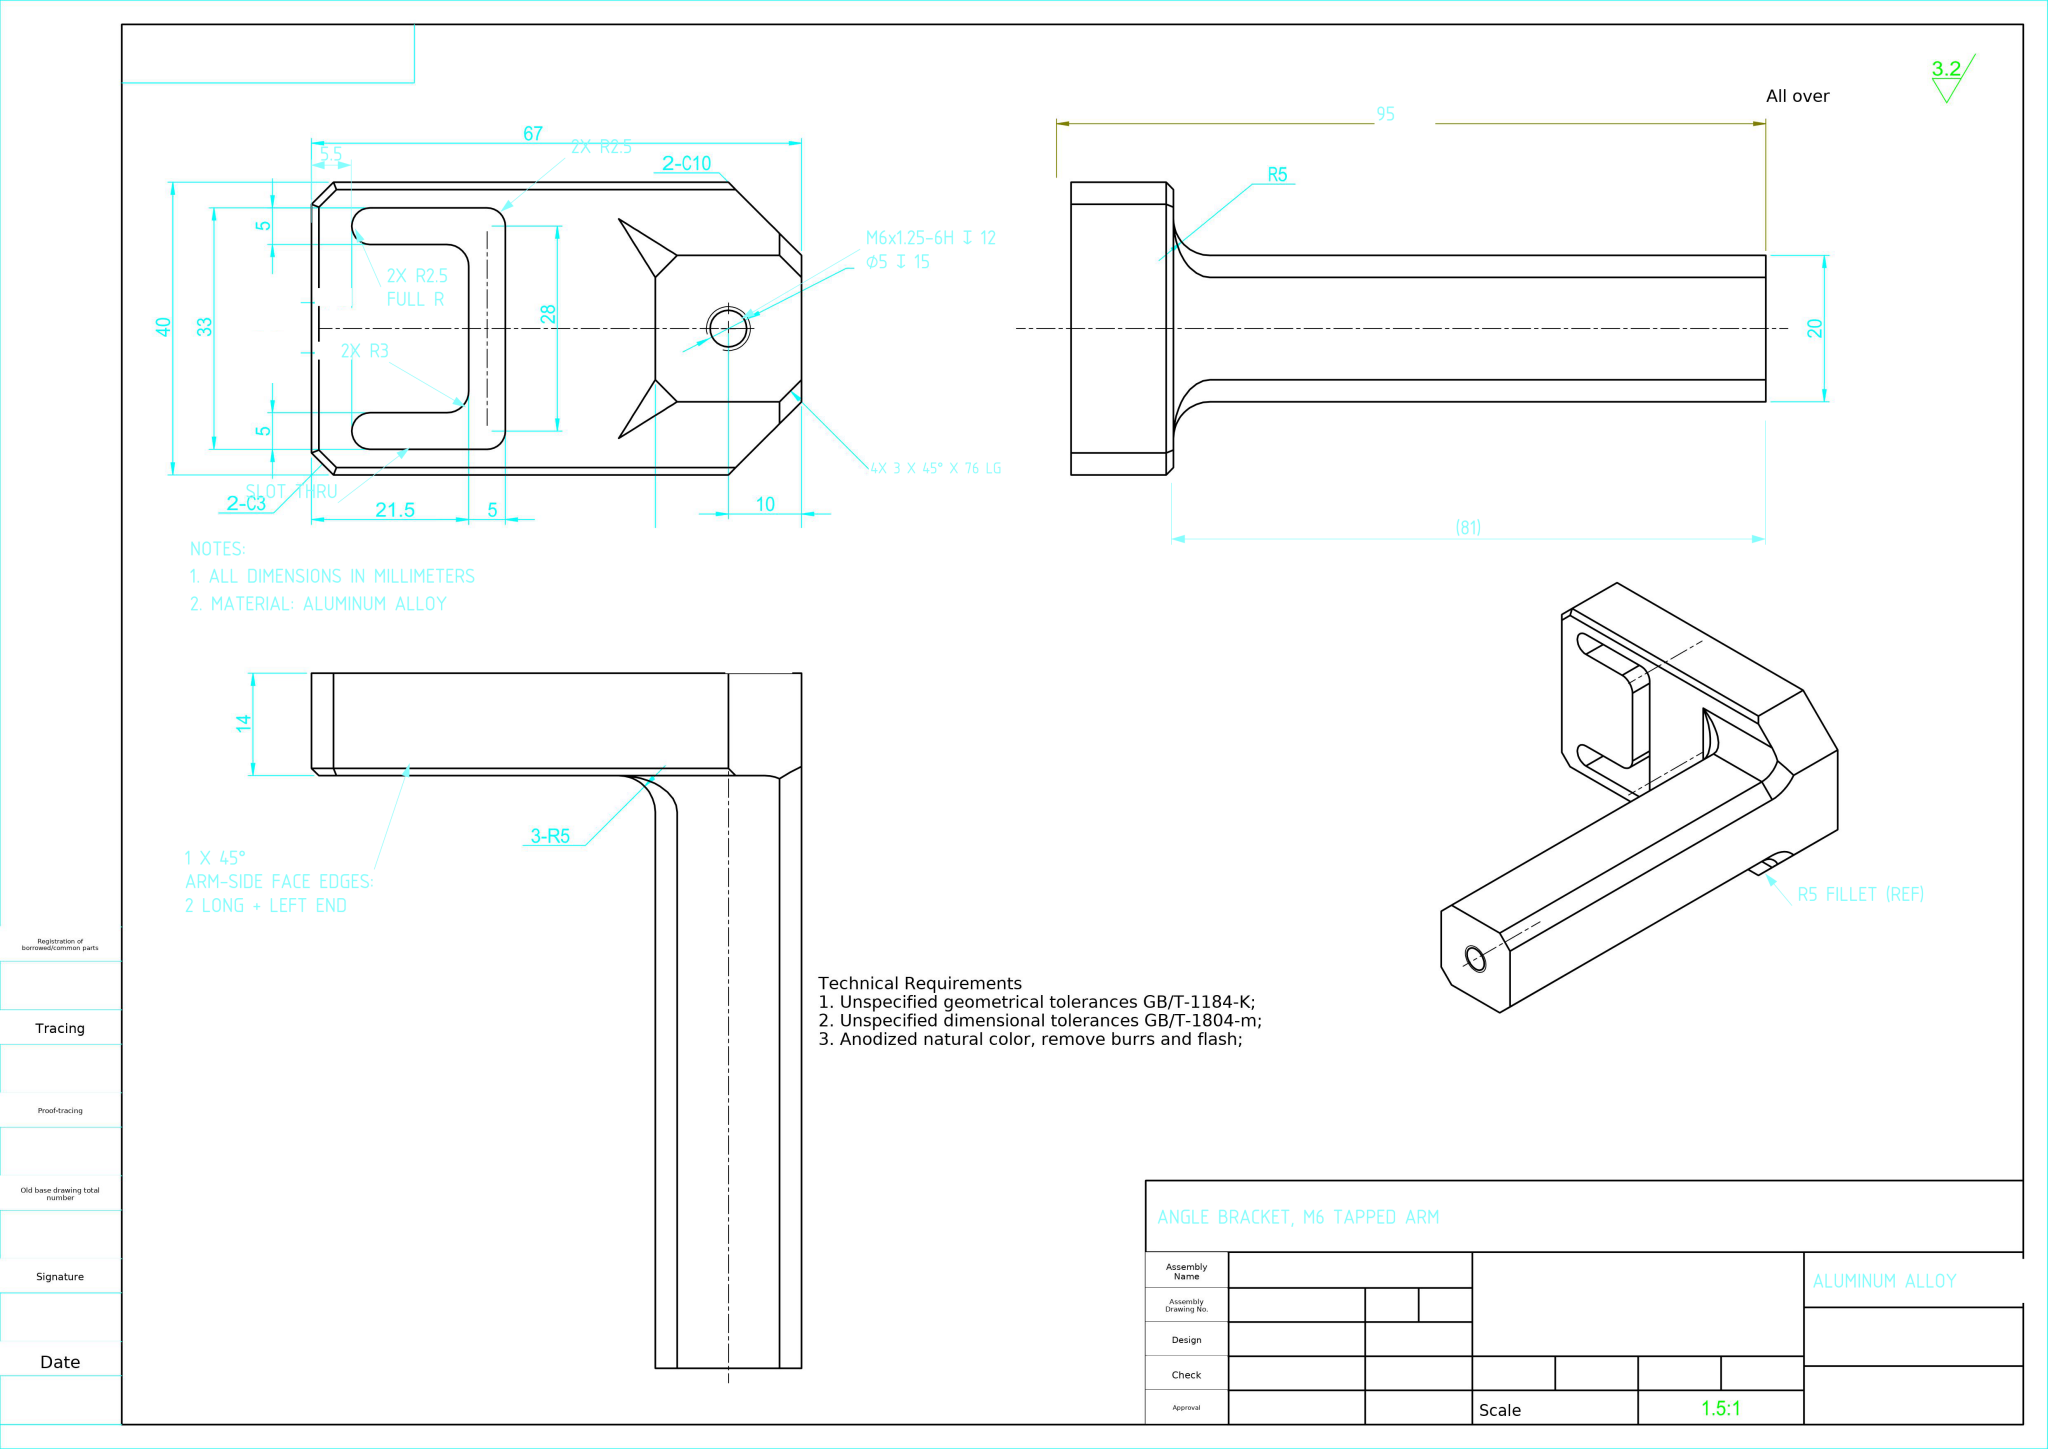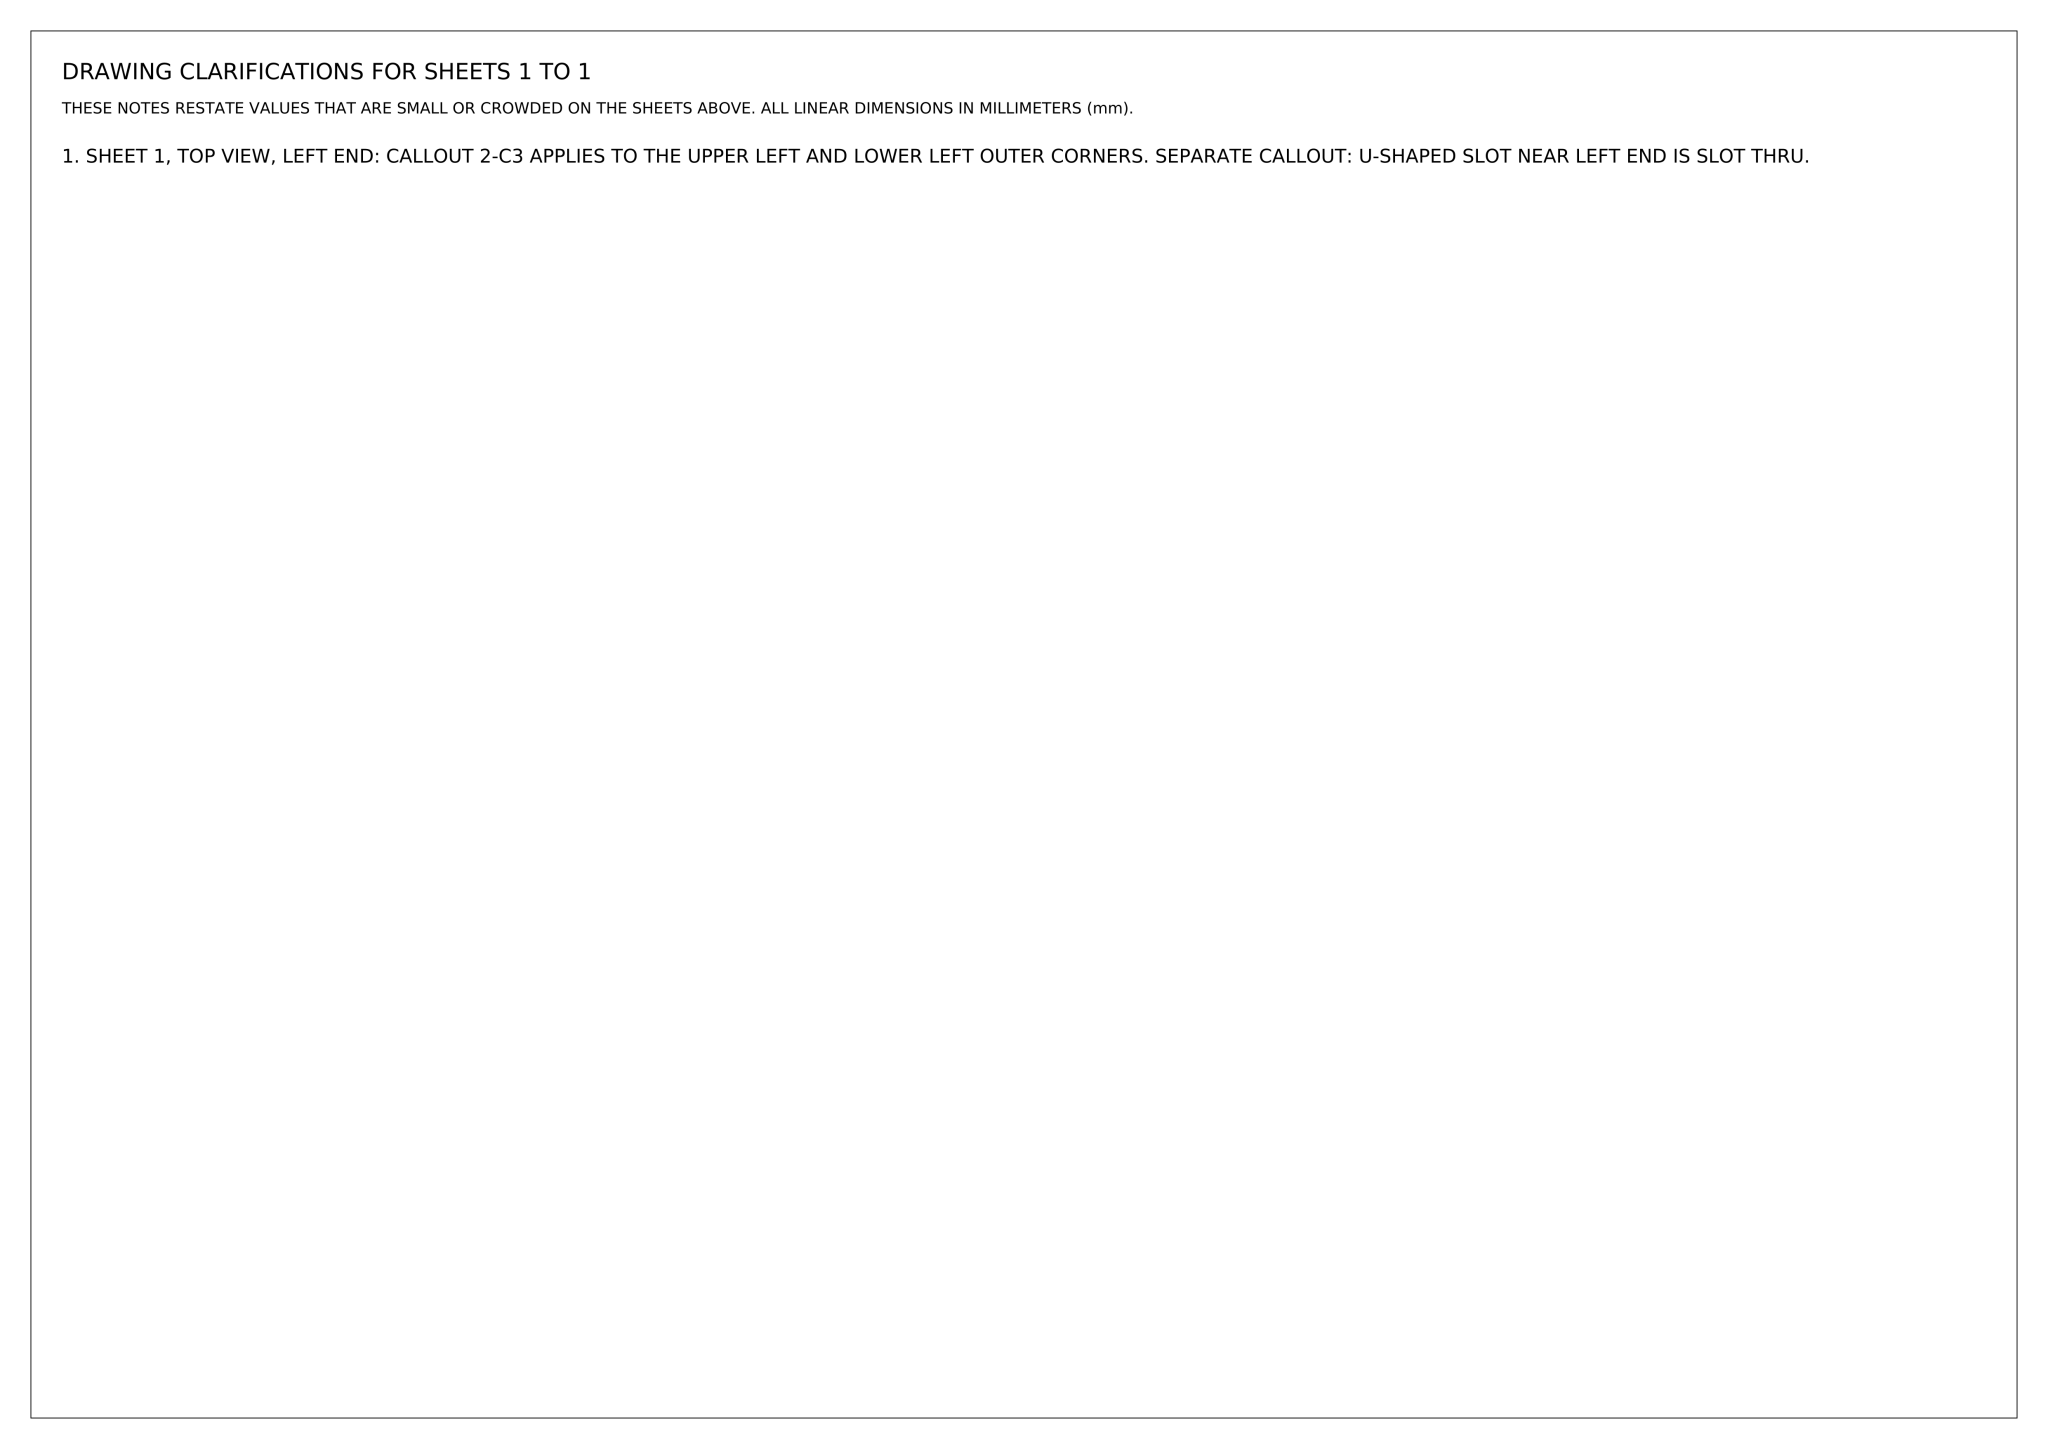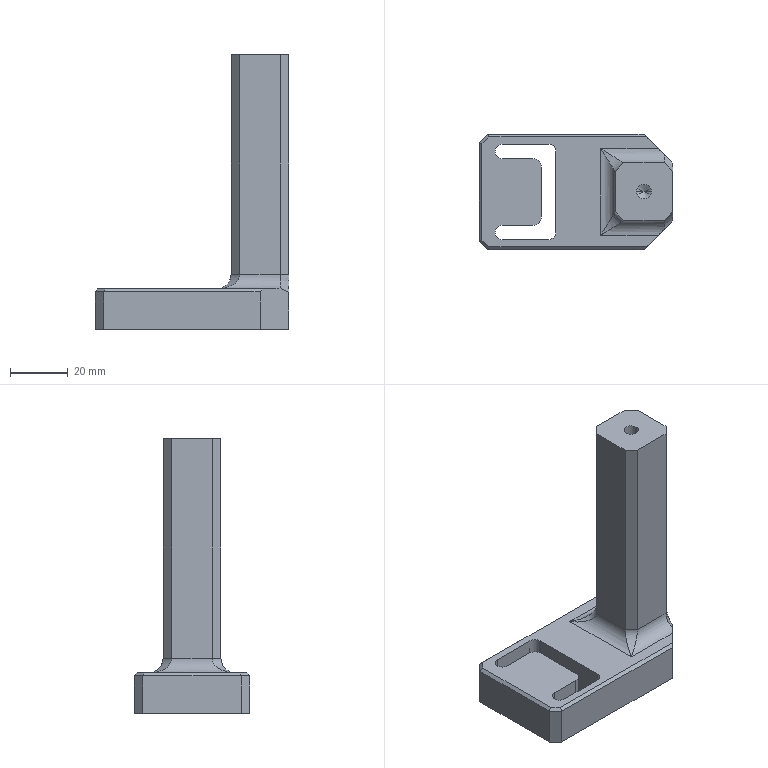Part | NX | mm | 1 solid | 46 faces | box 67 x 40 x 95 mm | volume 62413 mm3 | plane 29 | cylinder 11 | cone 4 | spline 2 | commonest cylinder face diameters 5 x6 10 x3 6 x2